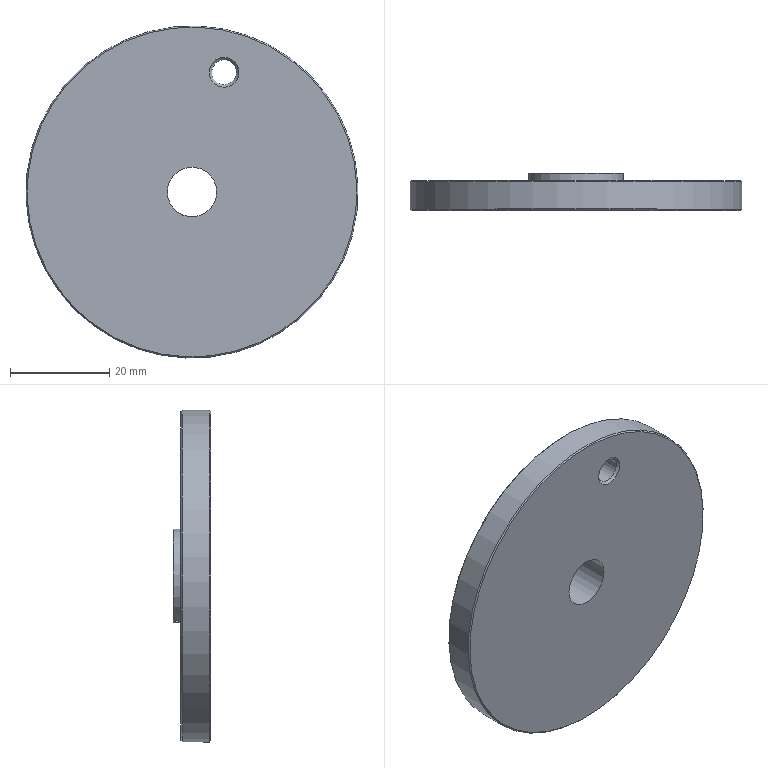Component | NX | CAM | 1 solid | 12 faces | volume 20852 mm3 | cylinder 5 | cone 4 | plane 3 | commonest cylinder face diameters 19 x1 10 x1 67 x1 5 x1 1 x1